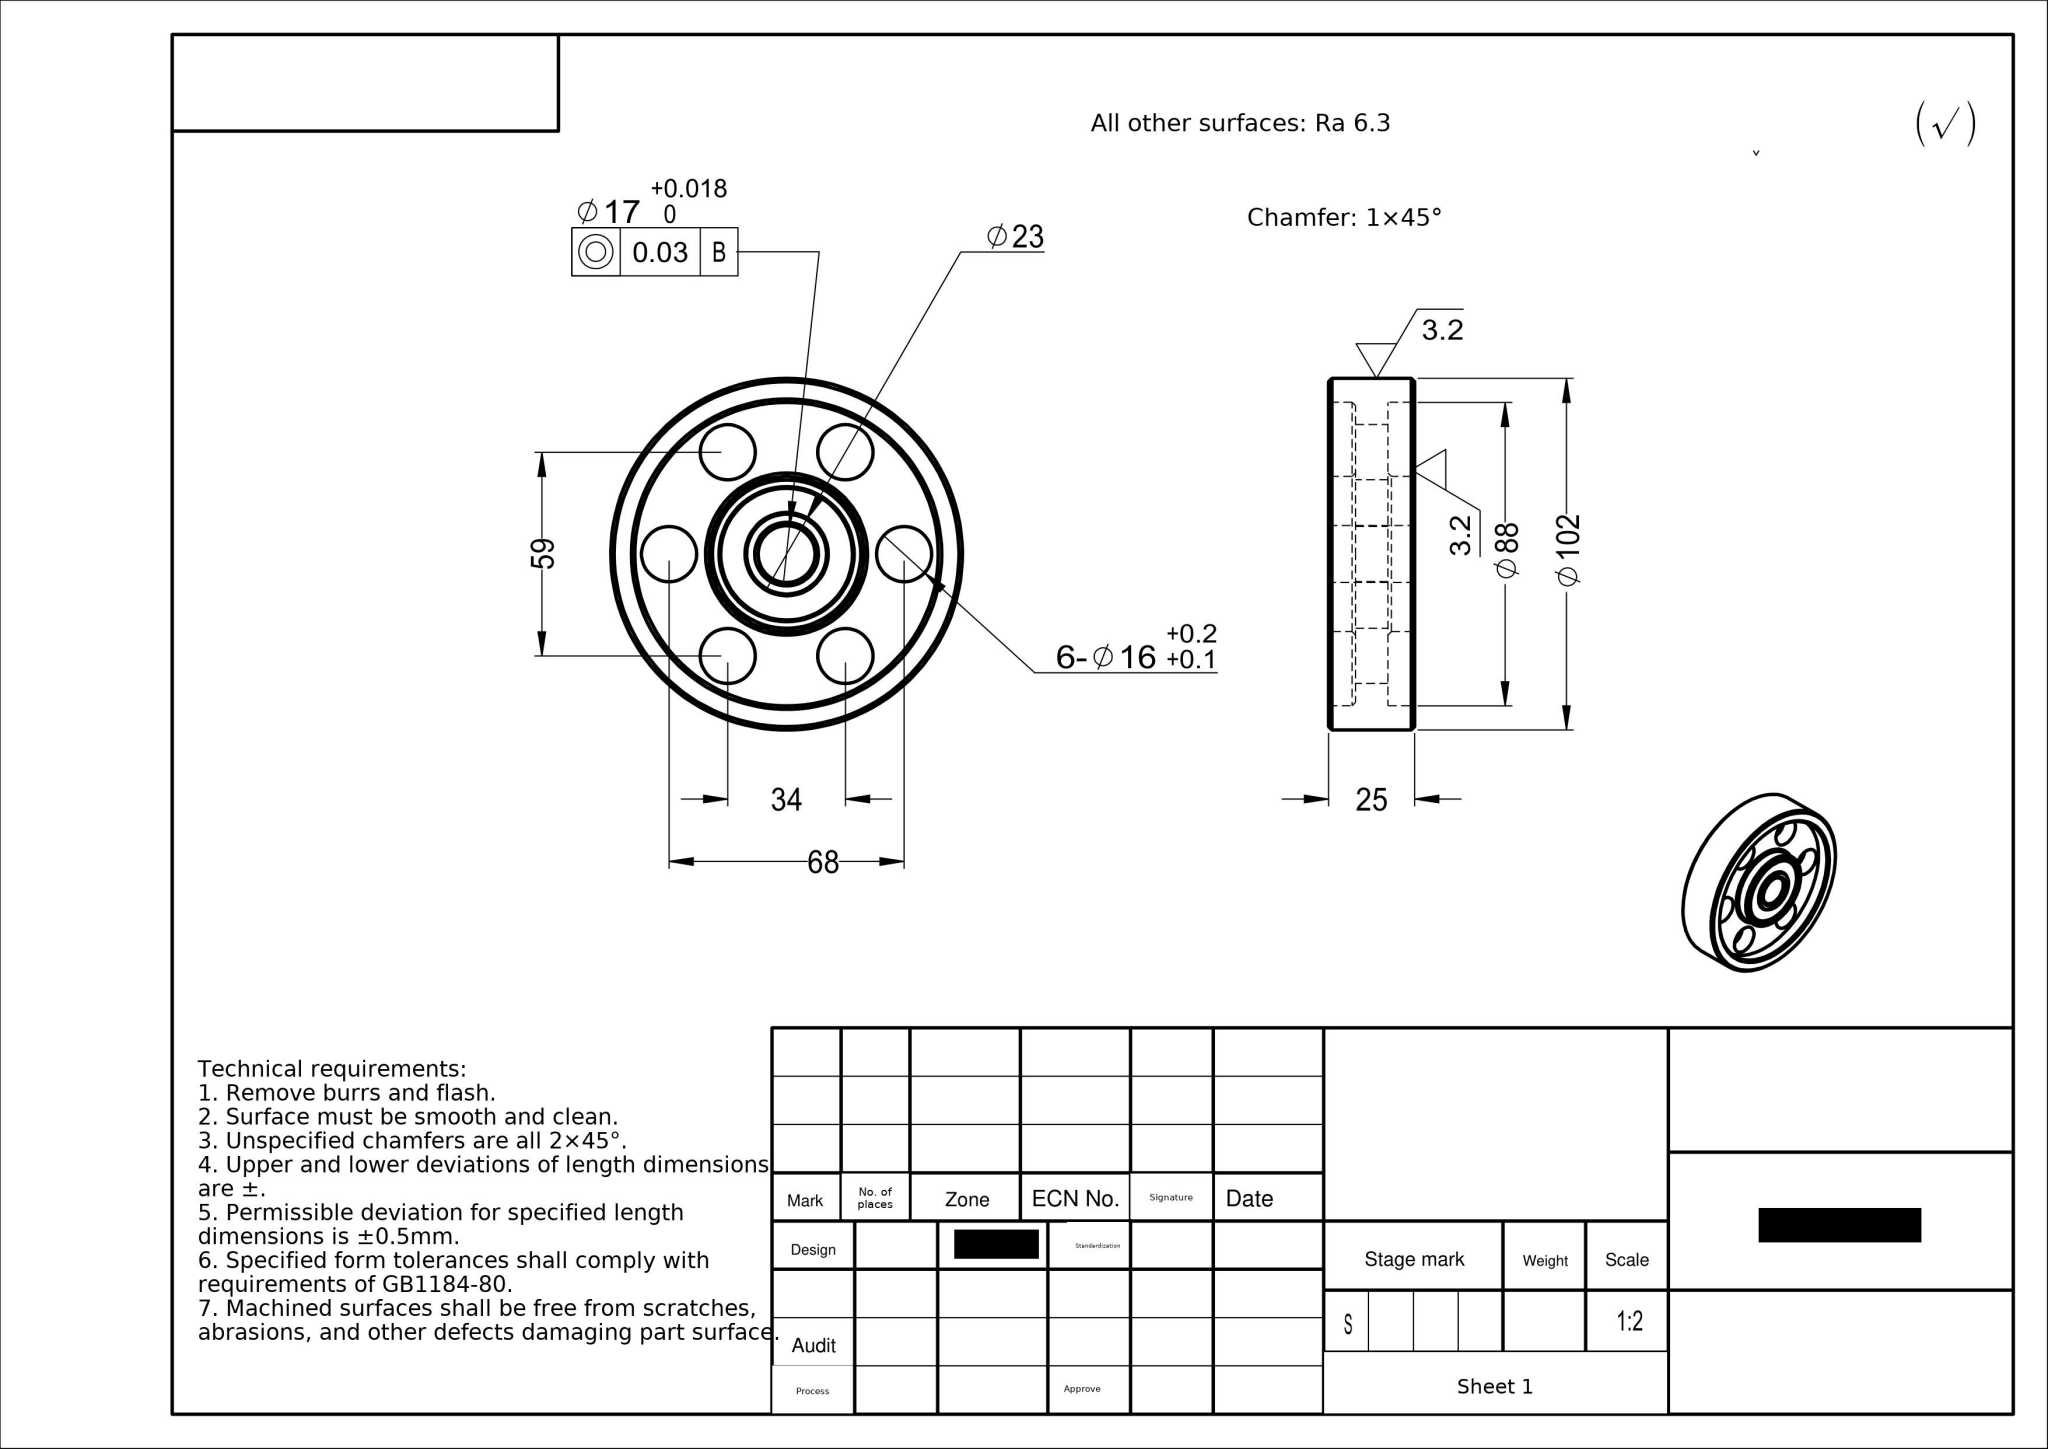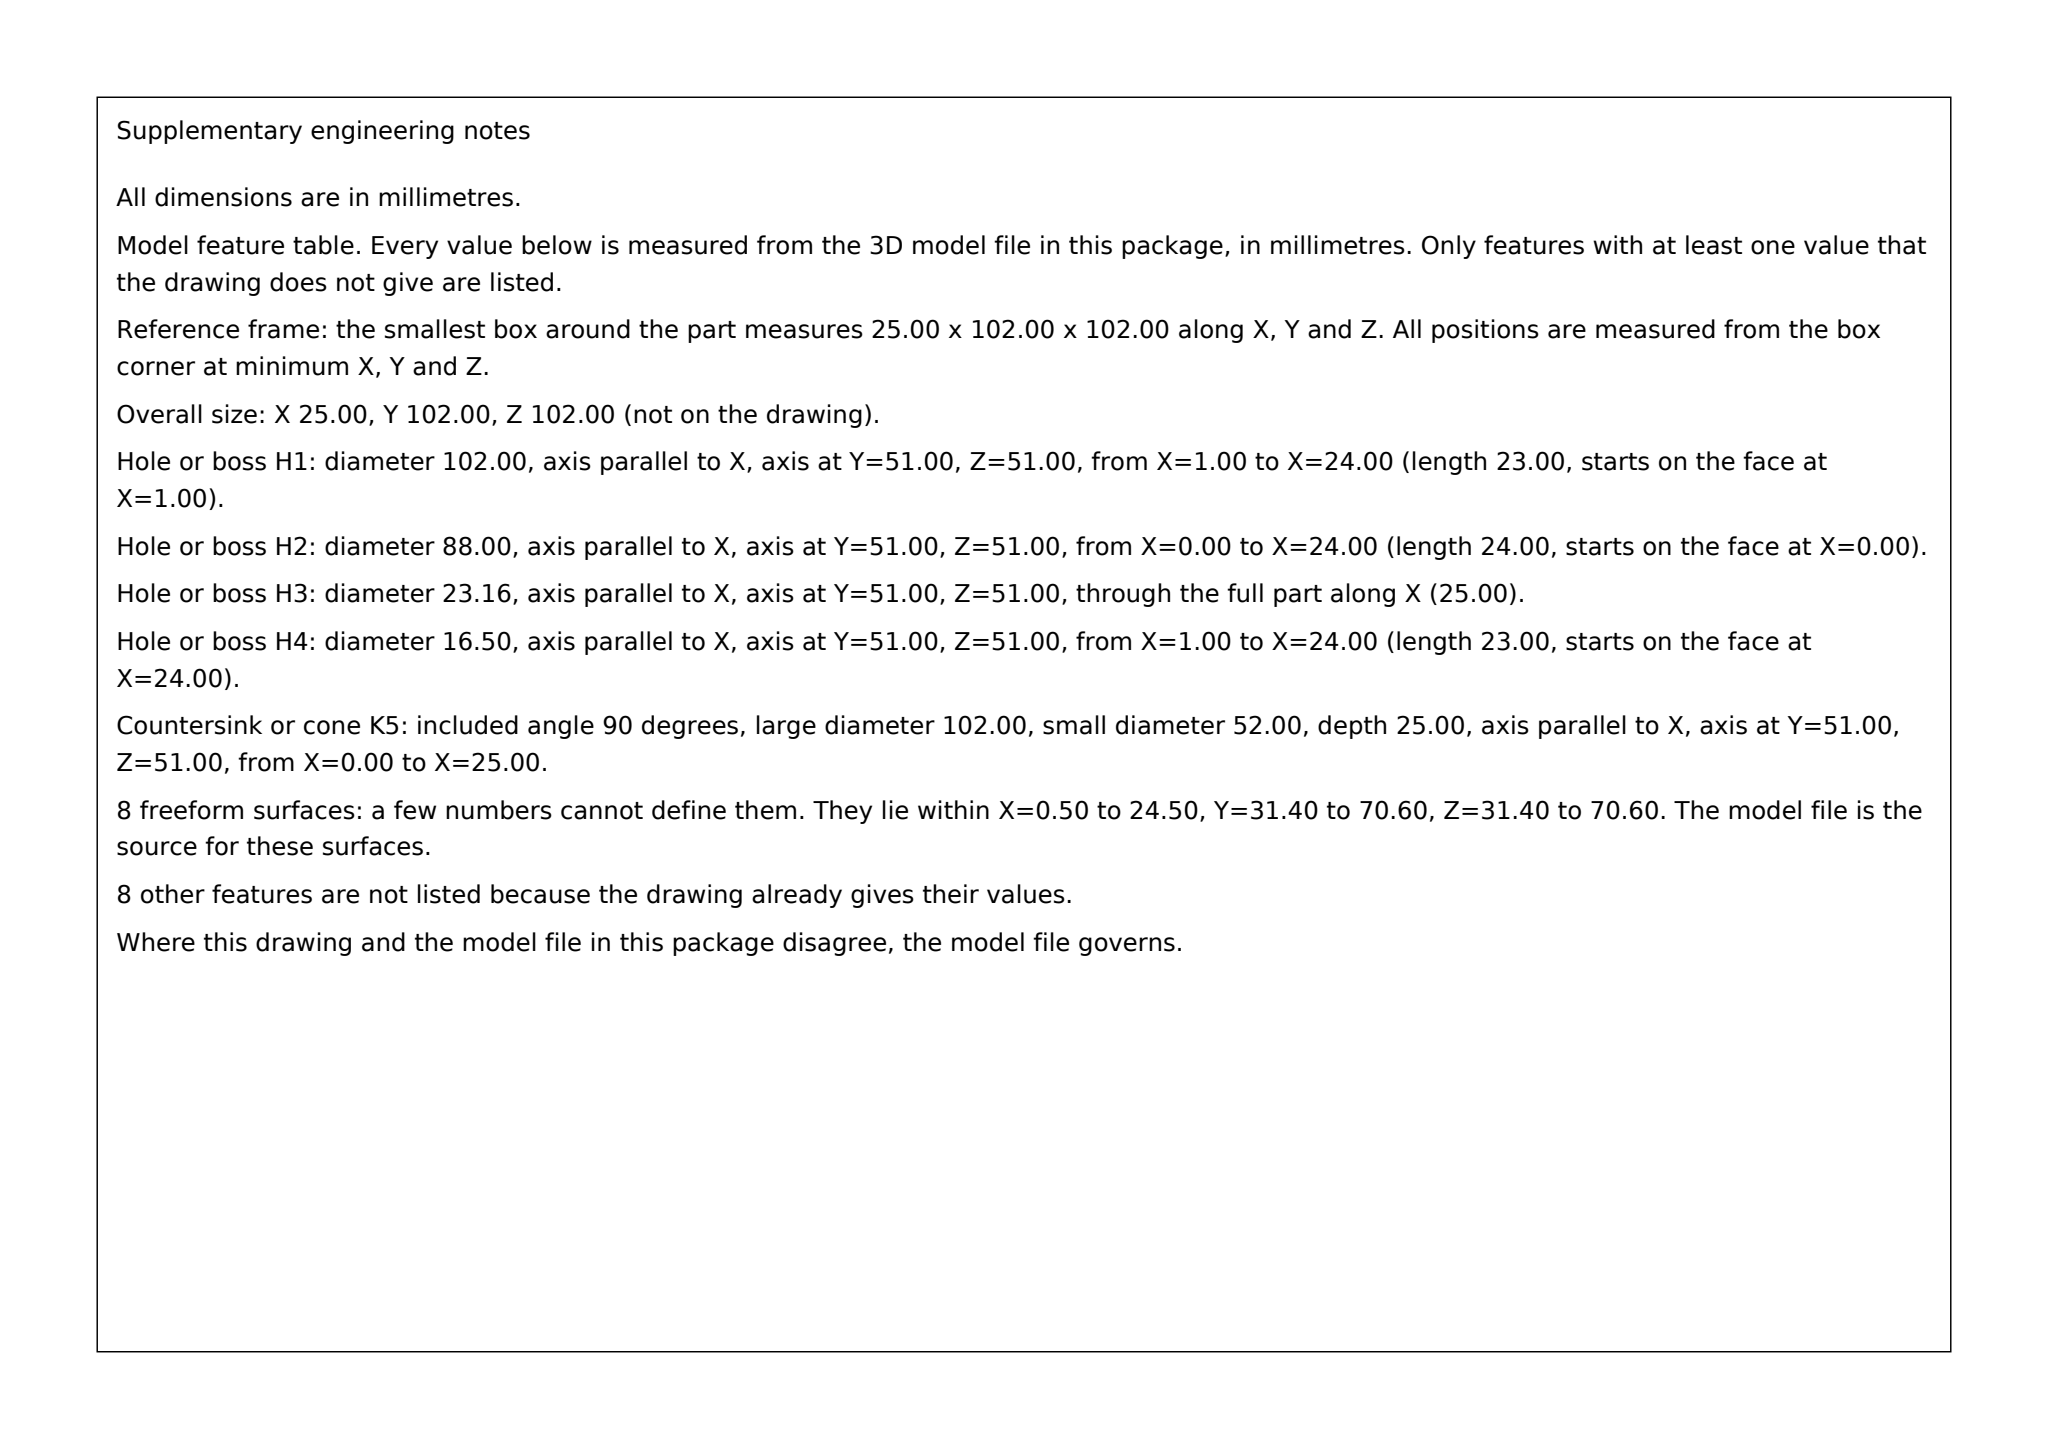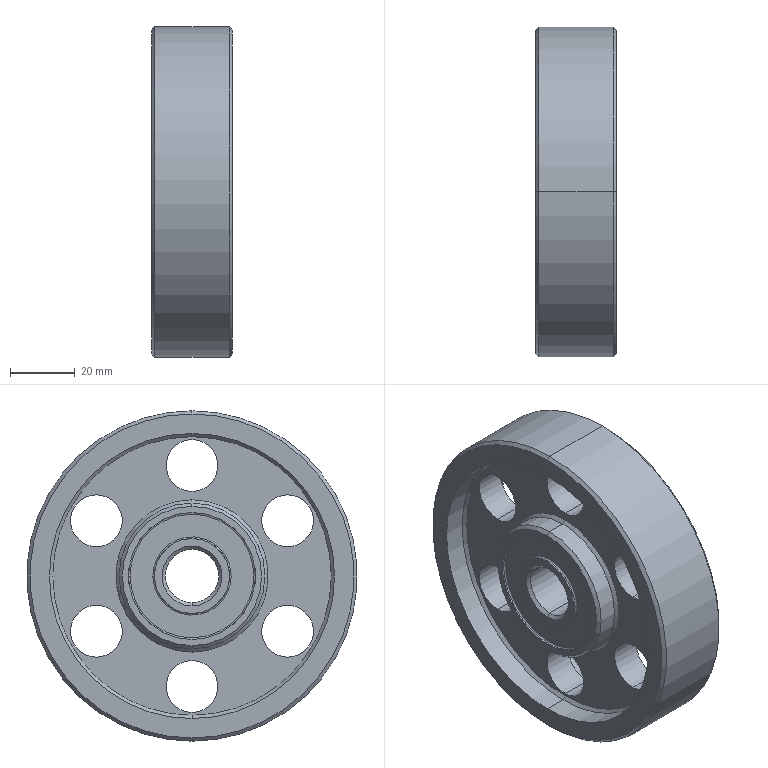Part | SolidWorks | mm | 1 solid | 70 faces | box 25 x 102 x 102 mm | volume 115598 mm3 | cylinder 32 | cone 20 | plane 10 | spline 8 | commonest cylinder face diameters 16 x12 88 x4 45 x4 39.208 x4 23.164 x4 102 x2 16.5 x2